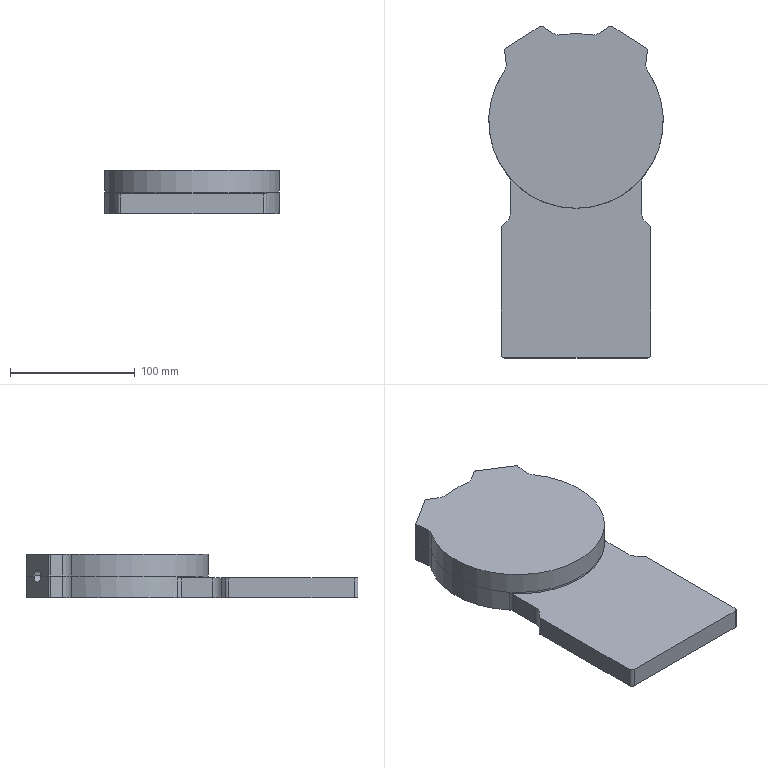CAM job | NX | mm | 3-axis | 2 set-ups | 6 operations | part box 140 x 266.17 x 35
set-up 1
1. Face Milling | Mill Mill5 D80 | FACE_MILLING | path 5032.557 mm | 3.925 min
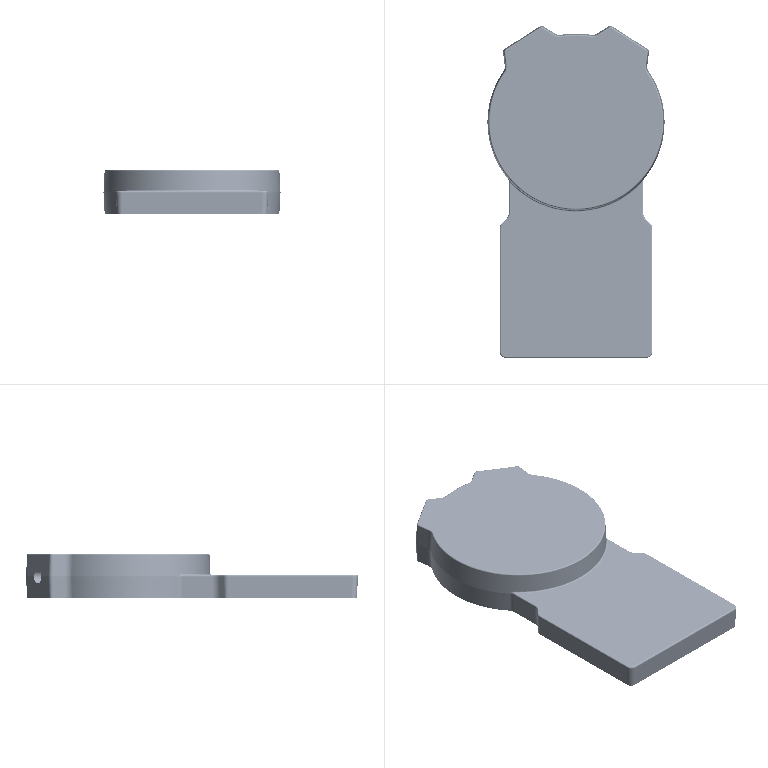2. Planar Milling | Mill Mill5 D10 | PLANAR_MILL | path 10534.774 mm | 6.935 min
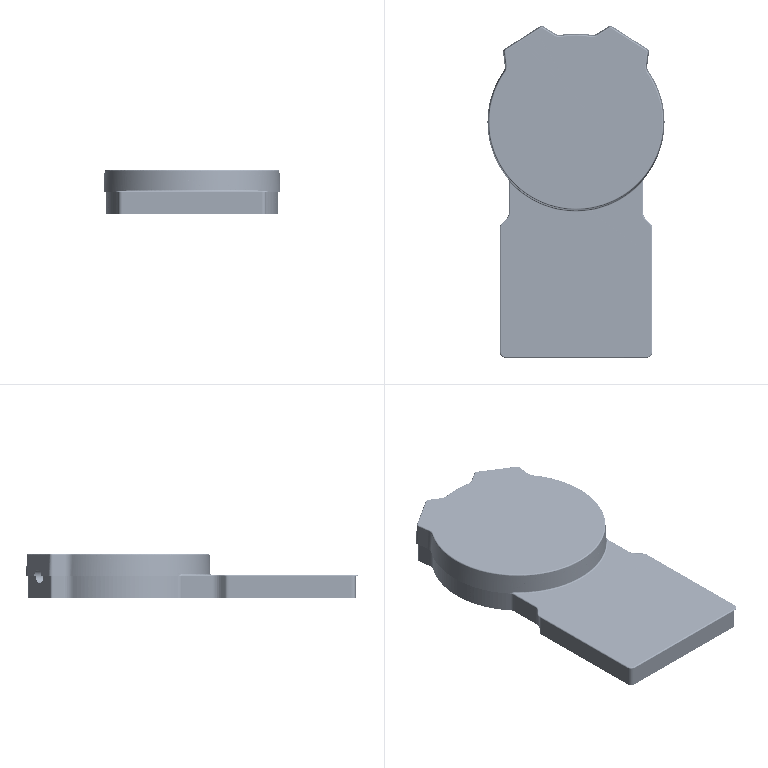3. Planar Milling | Mill Mill5 D10 | PLANAR_MILL_1 | path 860.68 mm | 0.7172 min
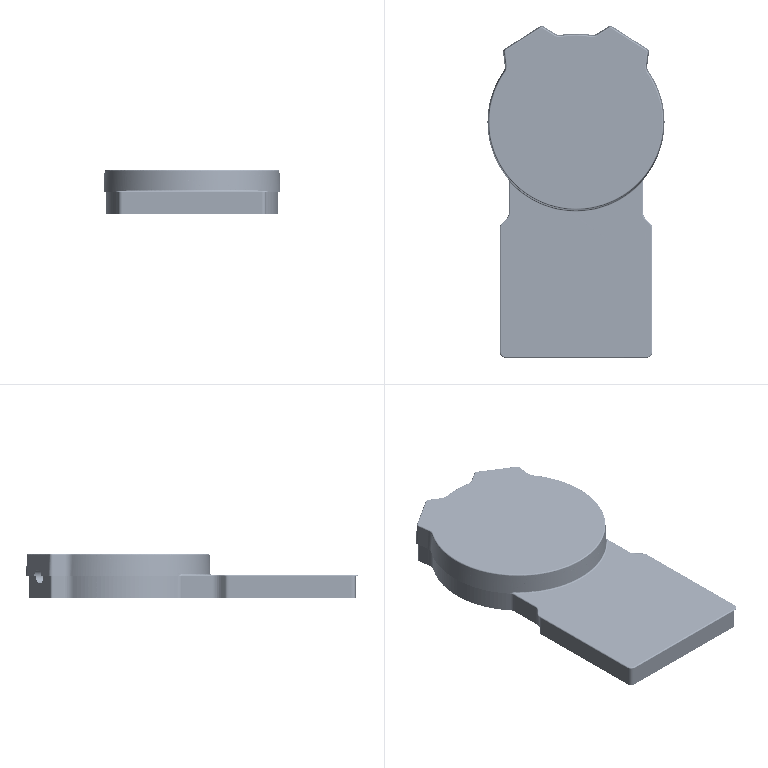set-up 2
4. Face Milling | Mill Mill5 D80 | FACE_MILLING_1 | path 3452.492 mm | 2.322 min
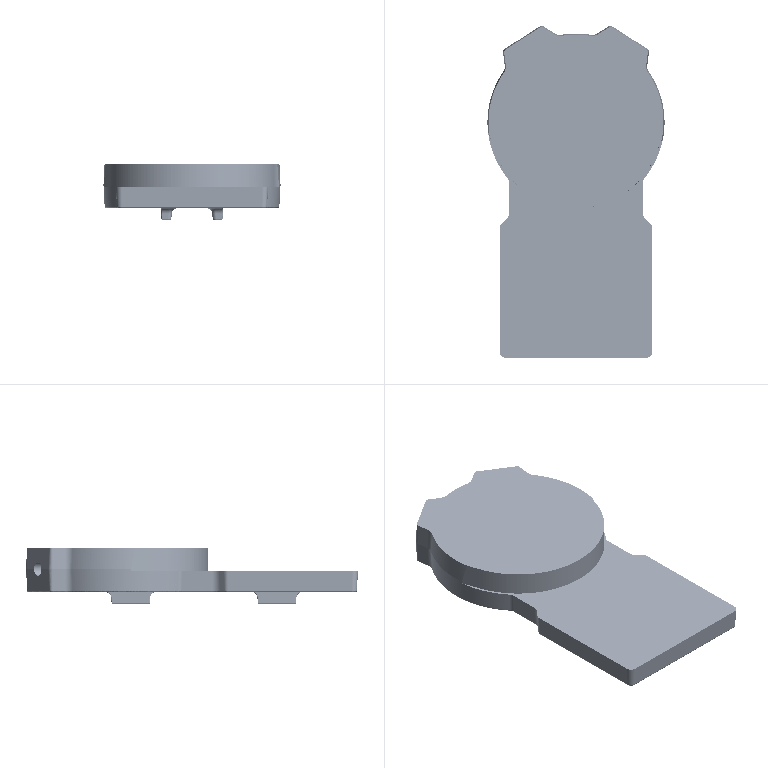5. Planar Milling | Mill Mill5 D10 | PLANAR_MILL_2 | path 6673.648 mm | 4.408 min
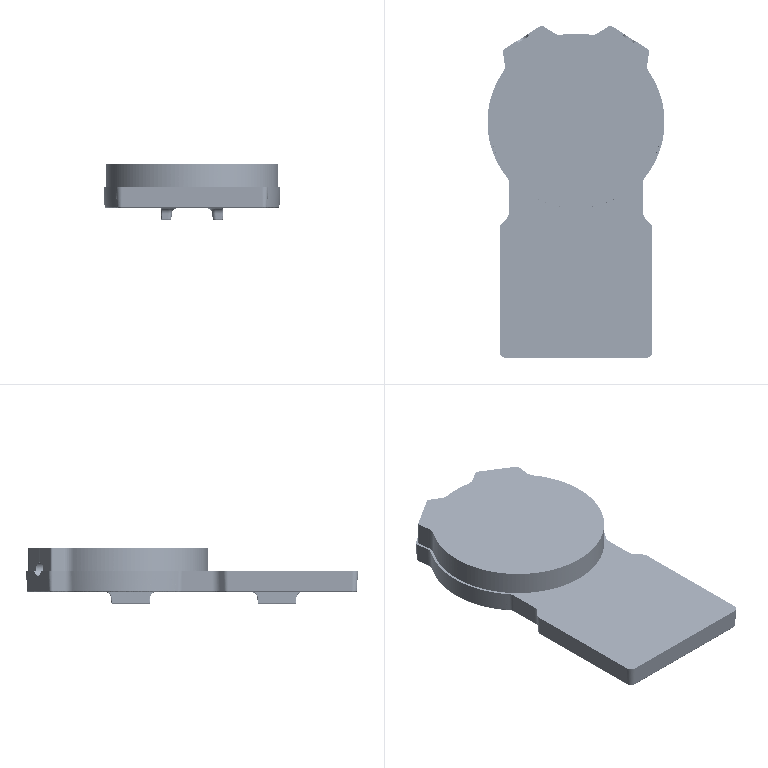6. Planar Milling | Mill Mill5 D10 | PLANAR_MILL_2_COPY | path 647.804 mm | 0.487 min